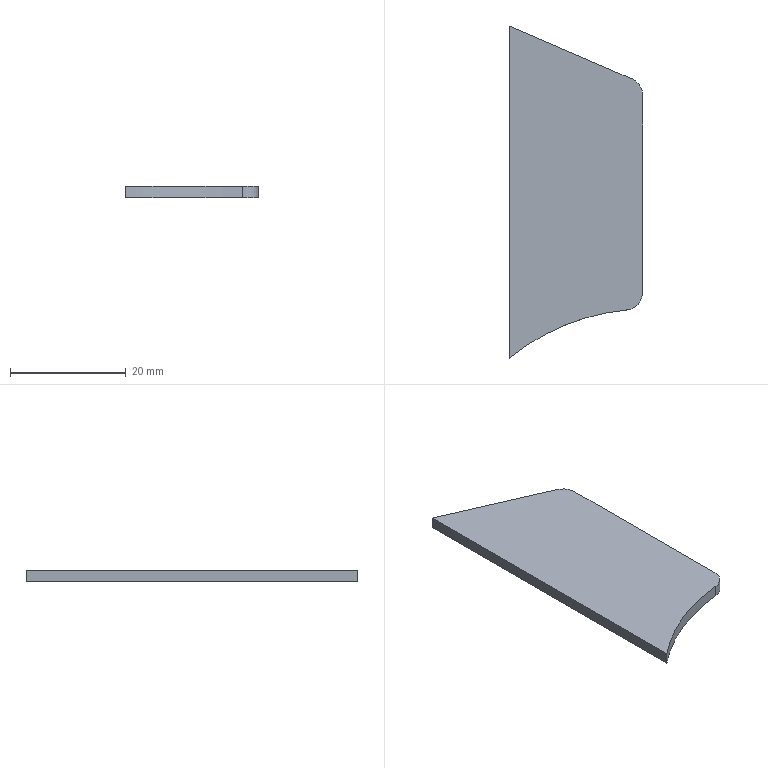Component | SolidWorks | YarnOutletAssembly-2_CashDispenserNozzleSidePlate-1 | 1 solid | 8 faces | box 23 x 57.4 x 2 mm | volume 2146 mm3 | plane 5 | cylinder 3 | commonest cylinder face diameters 6 x2 76 x1
STEP:
#1=COLOUR_RGB('',0.7922,0.8196,0.9333);
#2=FILL_AREA_STYLE_COLOUR('',#1);
#3=FILL_AREA_STYLE('',(#2));
#4=SURFACE_STYLE_FILL_AREA(#3);
#5=SURFACE_SIDE_STYLE('',(#4));
#6=SURFACE_STYLE_USAGE(.BOTH.,#5);
#7=PRESENTATION_STYLE_ASSIGNMENT((#6));
#8=CARTESIAN_POINT('',(-1.655,-15.942,-4.606));
#9=VERTEX_POINT('',#8);
#10=CARTESIAN_POINT('',(-1.655,-18.202,-4.606));
#11=VERTEX_POINT('',#10);
#12=CARTESIAN_POINT('',(-1.655,-18.202,-4.606));
#13=DIRECTION('',(0.,-1.,0.));
#14=VECTOR('',#13,39.37);
#15=LINE('',#12,#14);
#16=EDGE_CURVE('',#9,#11,#15,.T.);
#17=ORIENTED_EDGE('',*,*,#16,.F.);
#18=CARTESIAN_POINT('',(-1.655,-15.942,-4.685));
#19=VERTEX_POINT('',#18);
#20=CARTESIAN_POINT('',(-1.655,-15.942,-4.685));
#21=DIRECTION('',(-0.,0.,1.));
#22=VECTOR('',#21,39.37);
#23=LINE('',#20,#22);
#24=EDGE_CURVE('',#19,#9,#23,.T.);
#25=ORIENTED_EDGE('',*,*,#24,.F.);
#26=CARTESIAN_POINT('',(-1.655,-18.202,-4.685));
#27=VERTEX_POINT('',#26);
#28=CARTESIAN_POINT('',(-1.655,-18.202,-4.685));
#29=DIRECTION('',(0.,-1.,0.));
#30=VECTOR('',#29,39.37);
#31=LINE('',#28,#30);
#32=EDGE_CURVE('',#19,#27,#31,.T.);
#33=ORIENTED_EDGE('',*,*,#32,.T.);
#34=CARTESIAN_POINT('',(-1.655,-18.202,-4.685));
#35=DIRECTION('',(-0.,0.,1.));
#36=VECTOR('',#35,39.37);
#37=LINE('',#34,#36);
#38=EDGE_CURVE('',#27,#11,#37,.T.);
#39=ORIENTED_EDGE('',*,*,#38,.T.);
#40=EDGE_LOOP('',(#17,#25,#33,#39));
#41=FACE_OUTER_BOUND('',#40,.T.);
#42=CARTESIAN_POINT('',(-1.655,-18.202,-4.685));
#43=DIRECTION('',(-1.,-0.,-0.));
#44=DIRECTION('',(0.,-0.,-1.));
#45=AXIS2_PLACEMENT_3D('',#42,#43,#44);
#46=PLANE('',#45);
#47=ADVANCED_FACE('',(#41),#46,.T.);
#48=CARTESIAN_POINT('',(-0.8206,-16.302,-4.606));
#49=VERTEX_POINT('',#48);
#50=CARTESIAN_POINT('',(-1.655,-15.942,-4.606));
#51=DIRECTION('',(-0.918,0.3966,-0.));
#52=VECTOR('',#51,39.37);
#53=LINE('',#50,#52);
#54=EDGE_CURVE('',#49,#9,#53,.T.);
#55=ORIENTED_EDGE('',*,*,#54,.F.);
#56=CARTESIAN_POINT('',(-0.8206,-16.302,-4.685));
#57=VERTEX_POINT('',#56);
#58=CARTESIAN_POINT('',(-0.8206,-16.302,-4.685));
#59=DIRECTION('',(-0.,0.,1.));
#60=VECTOR('',#59,39.37);
#61=LINE('',#58,#60);
#62=EDGE_CURVE('',#57,#49,#61,.T.);
#63=ORIENTED_EDGE('',*,*,#62,.F.);
#64=CARTESIAN_POINT('',(-1.655,-15.942,-4.685));
#65=DIRECTION('',(-0.918,0.3966,-0.));
#66=VECTOR('',#65,39.37);
#67=LINE('',#64,#66);
#68=EDGE_CURVE('',#57,#19,#67,.T.);
#69=ORIENTED_EDGE('',*,*,#68,.T.);
#70=ORIENTED_EDGE('',*,*,#24,.T.);
#71=EDGE_LOOP('',(#55,#63,#69,#70));
#72=FACE_OUTER_BOUND('',#71,.T.);
#73=CARTESIAN_POINT('',(-1.655,-15.942,-4.685));
#74=DIRECTION('',(0.3966,0.918,-0.));
#75=DIRECTION('',(-0.918,0.3966,-0.));
#76=AXIS2_PLACEMENT_3D('',#73,#74,#75);
#77=PLANE('',#76);
#78=ADVANCED_FACE('',(#72),#77,.T.);
#79=CARTESIAN_POINT('',(-0.7493,-16.411,-4.606));
#80=VERTEX_POINT('',#79);
#81=CARTESIAN_POINT('',(-0.8674,-16.411,-4.606));
#82=DIRECTION('',(-0.,0.,1.));
#83=DIRECTION('',(0.,-1.,0.));
#84=AXIS2_PLACEMENT_3D('',#81,#82,#83);
#85=CIRCLE('',#84,0.1181);
#86=EDGE_CURVE('',#80,#49,#85,.T.);
#87=ORIENTED_EDGE('',*,*,#86,.F.);
#88=CARTESIAN_POINT('',(-0.7493,-16.411,-4.685));
#89=VERTEX_POINT('',#88);
#90=CARTESIAN_POINT('',(-0.7493,-16.411,-4.685));
#91=DIRECTION('',(-0.,0.,1.));
#92=VECTOR('',#91,39.37);
#93=LINE('',#90,#92);
#94=EDGE_CURVE('',#89,#80,#93,.T.);
#95=ORIENTED_EDGE('',*,*,#94,.F.);
#96=CARTESIAN_POINT('',(-0.8674,-16.411,-4.685));
#97=DIRECTION('',(-0.,0.,1.));
#98=DIRECTION('',(0.,-1.,0.));
#99=AXIS2_PLACEMENT_3D('',#96,#97,#98);
#100=CIRCLE('',#99,0.1181);
#101=EDGE_CURVE('',#89,#57,#100,.T.);
#102=ORIENTED_EDGE('',*,*,#101,.T.);
#103=ORIENTED_EDGE('',*,*,#62,.T.);
#104=EDGE_LOOP('',(#87,#95,#102,#103));
#105=FACE_OUTER_BOUND('',#104,.T.);
#106=CARTESIAN_POINT('',(-0.8674,-16.411,-4.685));
#107=DIRECTION('',(-0.,0.,1.));
#108=DIRECTION('',(0.,-1.,0.));
#109=AXIS2_PLACEMENT_3D('',#106,#107,#108);
#110=CYLINDRICAL_SURFACE('',#109,0.1181);
#111=ADVANCED_FACE('',(#105),#110,.T.);
#112=CARTESIAN_POINT('',(-0.7493,-17.757,-4.606));
#113=VERTEX_POINT('',#112);
#114=CARTESIAN_POINT('',(-0.7493,-16.411,-4.606));
#115=DIRECTION('',(-0.,1.,-0.));
#116=VECTOR('',#115,39.37);
#117=LINE('',#114,#116);
#118=EDGE_CURVE('',#113,#80,#117,.T.);
#119=ORIENTED_EDGE('',*,*,#118,.F.);
#120=CARTESIAN_POINT('',(-0.7493,-17.757,-4.685));
#121=VERTEX_POINT('',#120);
#122=CARTESIAN_POINT('',(-0.7493,-17.757,-4.685));
#123=DIRECTION('',(-0.,0.,1.));
#124=VECTOR('',#123,39.37);
#125=LINE('',#122,#124);
#126=EDGE_CURVE('',#121,#113,#125,.T.);
#127=ORIENTED_EDGE('',*,*,#126,.F.);
#128=CARTESIAN_POINT('',(-0.7493,-16.411,-4.685));
#129=DIRECTION('',(-0.,1.,-0.));
#130=VECTOR('',#129,39.37);
#131=LINE('',#128,#130);
#132=EDGE_CURVE('',#121,#89,#131,.T.);
#133=ORIENTED_EDGE('',*,*,#132,.T.);
#134=ORIENTED_EDGE('',*,*,#94,.T.);
#135=EDGE_LOOP('',(#119,#127,#133,#134));
#136=FACE_OUTER_BOUND('',#135,.T.);
#137=CARTESIAN_POINT('',(-0.7493,-16.411,-4.685));
#138=DIRECTION('',(1.,0.,0.));
#139=DIRECTION('',(-0.,0.,1.));
#140=AXIS2_PLACEMENT_3D('',#137,#138,#139);
#141=PLANE('',#140);
#142=ADVANCED_FACE('',(#136),#141,.T.);
#143=CARTESIAN_POINT('',(-0.8561,-17.875,-4.606));
#144=VERTEX_POINT('',#143);
#145=CARTESIAN_POINT('',(-0.8674,-17.757,-4.606));
#146=DIRECTION('',(-0.,0.,1.));
#147=DIRECTION('',(0.,-1.,0.));
#148=AXIS2_PLACEMENT_3D('',#145,#146,#147);
#149=CIRCLE('',#148,0.1181);
#150=EDGE_CURVE('',#144,#113,#149,.T.);
#151=ORIENTED_EDGE('',*,*,#150,.F.);
#152=CARTESIAN_POINT('',(-0.8561,-17.875,-4.685));
#153=VERTEX_POINT('',#152);
#154=CARTESIAN_POINT('',(-0.8561,-17.875,-4.685));
#155=DIRECTION('',(-0.,0.,1.));
#156=VECTOR('',#155,39.37);
#157=LINE('',#154,#156);
#158=EDGE_CURVE('',#153,#144,#157,.T.);
#159=ORIENTED_EDGE('',*,*,#158,.F.);
#160=CARTESIAN_POINT('',(-0.8674,-17.757,-4.685));
#161=DIRECTION('',(-0.,0.,1.));
#162=DIRECTION('',(0.,-1.,0.));
#163=AXIS2_PLACEMENT_3D('',#160,#161,#162);
#164=CIRCLE('',#163,0.1181);
#165=EDGE_CURVE('',#153,#121,#164,.T.);
#166=ORIENTED_EDGE('',*,*,#165,.T.);
#167=ORIENTED_EDGE('',*,*,#126,.T.);
#168=EDGE_LOOP('',(#151,#159,#166,#167));
#169=FACE_OUTER_BOUND('',#168,.T.);
#170=CARTESIAN_POINT('',(-0.8674,-17.757,-4.685));
#171=DIRECTION('',(-0.,0.,1.));
#172=DIRECTION('',(0.,-1.,0.));
#173=AXIS2_PLACEMENT_3D('',#170,#171,#172);
#174=CYLINDRICAL_SURFACE('',#173,0.1181);
#175=ADVANCED_FACE('',(#169),#174,.T.);
#176=CARTESIAN_POINT('',(-0.7132,-19.364,-4.606));
#177=DIRECTION('',(0.,-0.,-1.));
#178=DIRECTION('',(0.,-1.,0.));
#179=AXIS2_PLACEMENT_3D('',#176,#177,#178);
#180=CIRCLE('',#179,1.496);
#181=EDGE_CURVE('',#11,#144,#180,.T.);
#182=ORIENTED_EDGE('',*,*,#181,.F.);
#183=ORIENTED_EDGE('',*,*,#38,.F.);
#184=CARTESIAN_POINT('',(-0.7132,-19.364,-4.685));
#185=DIRECTION('',(0.,-0.,-1.));
#186=DIRECTION('',(0.,-1.,0.));
#187=AXIS2_PLACEMENT_3D('',#184,#185,#186);
#188=CIRCLE('',#187,1.496);
#189=EDGE_CURVE('',#27,#153,#188,.T.);
#190=ORIENTED_EDGE('',*,*,#189,.T.);
#191=ORIENTED_EDGE('',*,*,#158,.T.);
#192=EDGE_LOOP('',(#182,#183,#190,#191));
#193=FACE_OUTER_BOUND('',#192,.T.);
#194=CARTESIAN_POINT('',(-0.7132,-19.364,-4.685));
#195=DIRECTION('',(-0.,0.,1.));
#196=DIRECTION('',(0.,-1.,0.));
#197=AXIS2_PLACEMENT_3D('',#194,#195,#196);
#198=CYLINDRICAL_SURFACE('',#197,1.496);
#199=ADVANCED_FACE('',(#193),#198,.F.);
#200=ORIENTED_EDGE('',*,*,#32,.F.);
#201=ORIENTED_EDGE('',*,*,#68,.F.);
#202=ORIENTED_EDGE('',*,*,#101,.F.);
#203=ORIENTED_EDGE('',*,*,#132,.F.);
#204=ORIENTED_EDGE('',*,*,#165,.F.);
#205=ORIENTED_EDGE('',*,*,#189,.F.);
#206=EDGE_LOOP('',(#200,#201,#202,#203,#204,#205));
#207=FACE_OUTER_BOUND('',#206,.T.);
#208=CARTESIAN_POINT('',(-0.8674,-16.411,-4.685));
#209=DIRECTION('',(-0.,0.,1.));
#210=DIRECTION('',(0.,-1.,0.));
#211=AXIS2_PLACEMENT_3D('',#208,#209,#210);
#212=PLANE('',#211);
#213=ADVANCED_FACE('',(#207),#212,.F.);
#214=ORIENTED_EDGE('',*,*,#16,.T.);
#215=ORIENTED_EDGE('',*,*,#181,.T.);
#216=ORIENTED_EDGE('',*,*,#150,.T.);
#217=ORIENTED_EDGE('',*,*,#118,.T.);
#218=ORIENTED_EDGE('',*,*,#86,.T.);
#219=ORIENTED_EDGE('',*,*,#54,.T.);
#220=EDGE_LOOP('',(#214,#215,#216,#217,#218,#219));
#221=FACE_OUTER_BOUND('',#220,.T.);
#222=CARTESIAN_POINT('',(-0.8674,-16.411,-4.606));
#223=DIRECTION('',(-0.,0.,1.));
#224=DIRECTION('',(0.,-1.,0.));
#225=AXIS2_PLACEMENT_3D('',#222,#223,#224);
#226=PLANE('',#225);
#227=ADVANCED_FACE('',(#221),#226,.T.);
#228=CLOSED_SHELL('',(#47,#78,#111,#142,#175,#199,#213,#227));
#229=MANIFOLD_SOLID_BREP('',#228);
#230=STYLED_ITEM('',(#7),#229);
#231=(LENGTH_UNIT()NAMED_UNIT(*)SI_UNIT($,.METRE.));
#232=LENGTH_MEASURE_WITH_UNIT(LENGTH_MEASURE(0.0254),#231);
#233=DIMENSIONAL_EXPONENTS(1.,0.,0.,0.,0.,0.,0.);
#234=(CONVERSION_BASED_UNIT('',#232)LENGTH_UNIT()NAMED_UNIT(#233));
#235=UNCERTAINTY_MEASURE_WITH_UNIT(LENGTH_MEASURE(0.00001),#234,'','');
#236=(NAMED_UNIT(*)PLANE_ANGLE_UNIT()SI_UNIT($,.RADIAN.));
#237=(NAMED_UNIT(*)SI_UNIT($,.STERADIAN.)SOLID_ANGLE_UNIT());
#238=(GEOMETRIC_REPRESENTATION_CONTEXT(3)GLOBAL_UNCERTAINTY_ASSIGNED_CONTEXT((#235))GLOBAL_UNIT_ASSIGNED_CONTEXT((#234,#236,#237))REPRESENTATION_CONTEXT('',''));
#239=MECHANICAL_DESIGN_GEOMETRIC_PRESENTATION_REPRESENTATION('',(#230),#238);
#240=CARTESIAN_POINT('',(0.,0.,0.));
#241=DIRECTION('',(0.,0.,1.));
#242=DIRECTION('',(1.,0.,0.));
#243=AXIS2_PLACEMENT_3D('',#240,#241,#242);
#244=(LENGTH_UNIT()NAMED_UNIT(*)SI_UNIT($,.METRE.));
#245=LENGTH_MEASURE_WITH_UNIT(LENGTH_MEASURE(0.0254),#244);
#246=DIMENSIONAL_EXPONENTS(1.,0.,0.,0.,0.,0.,0.);
#247=(CONVERSION_BASED_UNIT('',#245)LENGTH_UNIT()NAMED_UNIT(#246));
#248=UNCERTAINTY_MEASURE_WITH_UNIT(LENGTH_MEASURE(0.00001),#247,'','');
#249=(NAMED_UNIT(*)PLANE_ANGLE_UNIT()SI_UNIT($,.RADIAN.));
#250=(NAMED_UNIT(*)SI_UNIT($,.STERADIAN.)SOLID_ANGLE_UNIT());
#251=(GEOMETRIC_REPRESENTATION_CONTEXT(3)GLOBAL_UNCERTAINTY_ASSIGNED_CONTEXT((#248))GLOBAL_UNIT_ASSIGNED_CONTEXT((#247,#249,#250))REPRESENTATION_CONTEXT('',''));
#252=ADVANCED_BREP_SHAPE_REPRESENTATION('',(#229,#243),#251);
#253=PRESENTATION_LAYER_ASSIGNMENT('','',(#230));